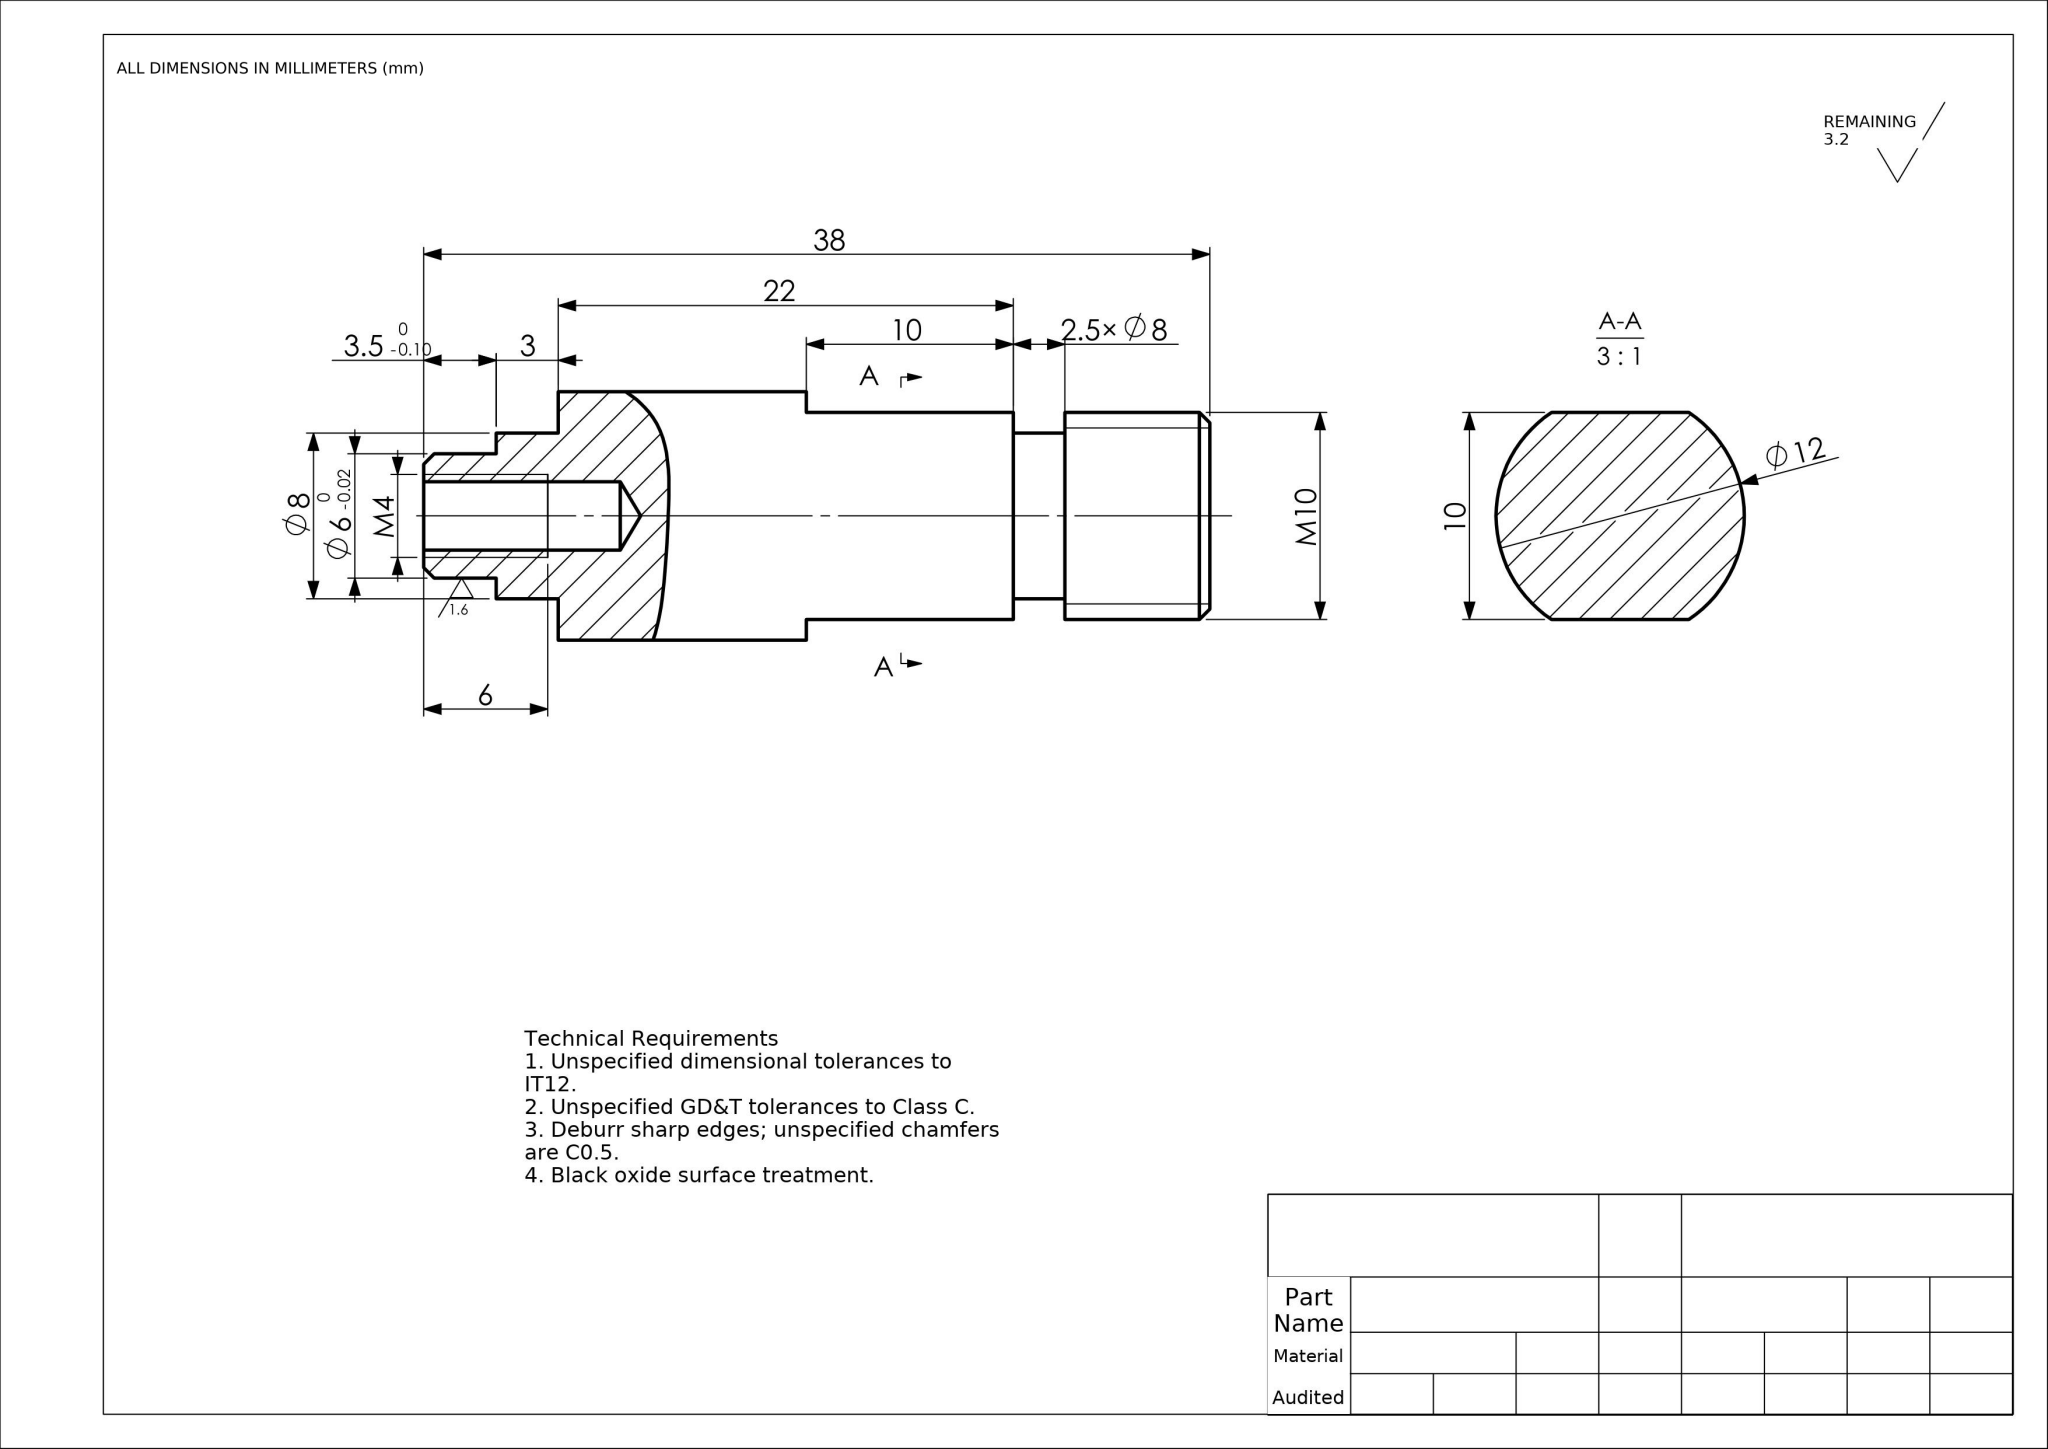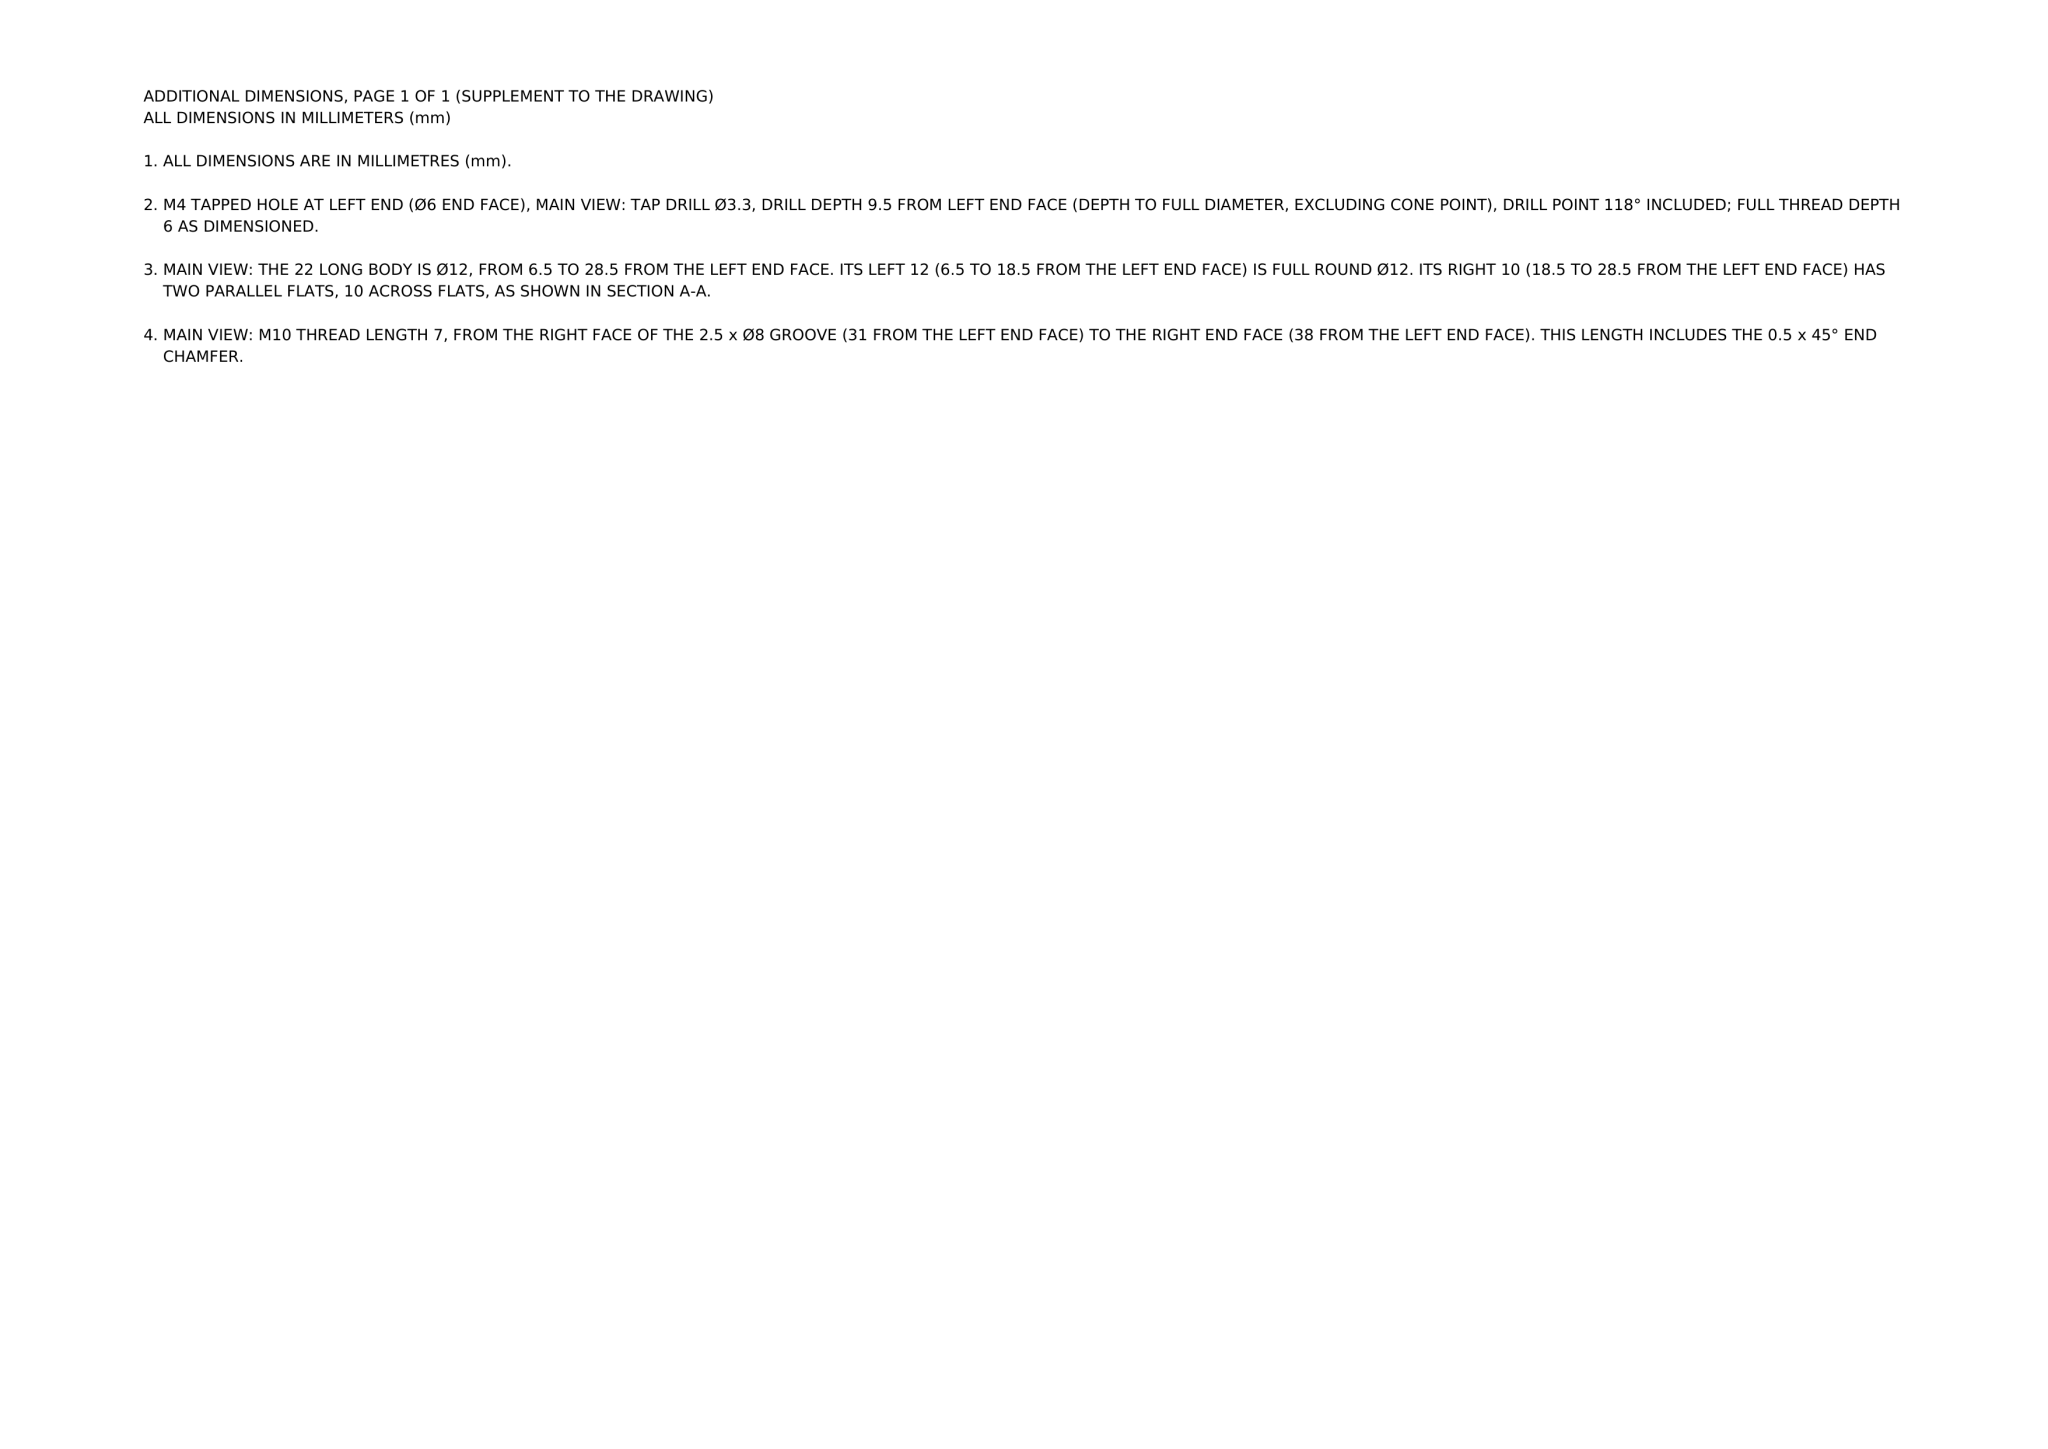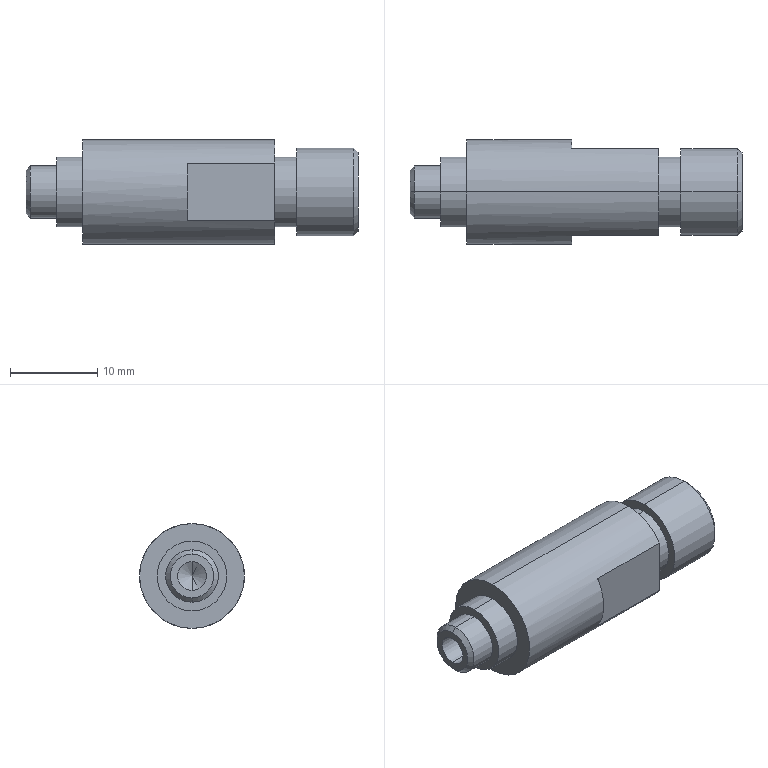Part | NX | mm | 1 solid | 28 faces | box 38 x 12 x 12 mm | volume 3233 mm3 | cylinder 12 | plane 10 | cone 6 | commonest cylinder face diameters 8 x4 3.3 x2 10 x2 12 x2 6 x2
STEP:
#1=COLOUR_RGB('',0.7961,0.8235,0.9373);
#2=FILL_AREA_STYLE_COLOUR('',#1);
#3=FILL_AREA_STYLE('',(#2));
#4=SURFACE_STYLE_FILL_AREA(#3);
#5=SURFACE_SIDE_STYLE('',(#4));
#6=SURFACE_STYLE_USAGE(.BOTH.,#5);
#7=PRESENTATION_STYLE_ASSIGNMENT((#6));
#8=CARTESIAN_POINT('',(9.5,0.,-1.65));
#9=VERTEX_POINT('',#8);
#10=CARTESIAN_POINT('',(9.5,0.,1.65));
#11=VERTEX_POINT('',#10);
#12=CARTESIAN_POINT('',(9.5,0.,0.));
#13=DIRECTION('',(-1.,0.,0.));
#14=DIRECTION('',(0.,0.,1.));
#15=AXIS2_PLACEMENT_3D('',#12,#13,#14);
#16=CIRCLE('',#15,1.65);
#17=EDGE_CURVE('',#9,#11,#16,.T.);
#18=ORIENTED_EDGE('',*,*,#17,.F.);
#19=CARTESIAN_POINT('',(-0.,0.,-1.65));
#20=VERTEX_POINT('',#19);
#21=CARTESIAN_POINT('',(0.,0.,-1.65));
#22=DIRECTION('',(-1.,0.,0.));
#23=VECTOR('',#22,1000.);
#24=LINE('',#21,#23);
#25=EDGE_CURVE('',#9,#20,#24,.T.);
#26=ORIENTED_EDGE('',*,*,#25,.T.);
#27=CARTESIAN_POINT('',(-0.,0.,1.65));
#28=VERTEX_POINT('',#27);
#29=CARTESIAN_POINT('',(-0.,0.,0.));
#30=DIRECTION('',(-1.,0.,0.));
#31=DIRECTION('',(0.,0.,1.));
#32=AXIS2_PLACEMENT_3D('',#29,#30,#31);
#33=CIRCLE('',#32,1.65);
#34=EDGE_CURVE('',#20,#28,#33,.T.);
#35=ORIENTED_EDGE('',*,*,#34,.T.);
#36=CARTESIAN_POINT('',(0.,0.,1.65));
#37=DIRECTION('',(-1.,0.,0.));
#38=VECTOR('',#37,1000.);
#39=LINE('',#36,#38);
#40=EDGE_CURVE('',#11,#28,#39,.T.);
#41=ORIENTED_EDGE('',*,*,#40,.F.);
#42=EDGE_LOOP('',(#18,#26,#35,#41));
#43=FACE_OUTER_BOUND('',#42,.T.);
#44=CARTESIAN_POINT('',(0.,0.,0.));
#45=DIRECTION('',(-1.,0.,0.));
#46=DIRECTION('',(0.,0.,1.));
#47=AXIS2_PLACEMENT_3D('',#44,#45,#46);
#48=CYLINDRICAL_SURFACE('',#47,1.65);
#49=ADVANCED_FACE('',(#43),#48,.F.);
#50=CARTESIAN_POINT('',(10.491,-0.,0.));
#51=VERTEX_POINT('',#50);
#52=CARTESIAN_POINT('',(9.5,0.,1.65));
#53=DIRECTION('',(-0.515,0.,0.8572));
#54=VECTOR('',#53,1000.);
#55=LINE('',#52,#54);
#56=EDGE_CURVE('',#51,#11,#55,.T.);
#57=ORIENTED_EDGE('',*,*,#56,.F.);
#58=CARTESIAN_POINT('',(9.5,0.,-1.65));
#59=DIRECTION('',(-0.515,0.,-0.8572));
#60=VECTOR('',#59,1000.);
#61=LINE('',#58,#60);
#62=EDGE_CURVE('',#51,#9,#61,.T.);
#63=ORIENTED_EDGE('',*,*,#62,.T.);
#64=ORIENTED_EDGE('',*,*,#17,.T.);
#65=EDGE_LOOP('',(#57,#63,#64));
#66=FACE_OUTER_BOUND('',#65,.T.);
#67=CARTESIAN_POINT('',(9.5,0.,0.));
#68=DIRECTION('',(-1.,0.,0.));
#69=DIRECTION('',(0.,0.,1.));
#70=AXIS2_PLACEMENT_3D('',#67,#68,#69);
#71=CONICAL_SURFACE('',#70,1.65,1.03);
#72=ADVANCED_FACE('',(#66),#71,.F.);
#73=CARTESIAN_POINT('',(0.,0.,2.5));
#74=VERTEX_POINT('',#73);
#75=CARTESIAN_POINT('',(0.,0.,-2.5));
#76=VERTEX_POINT('',#75);
#77=CARTESIAN_POINT('',(0.,0.,0.));
#78=DIRECTION('',(-1.,0.,0.));
#79=DIRECTION('',(0.,0.,-1.));
#80=AXIS2_PLACEMENT_3D('',#77,#78,#79);
#81=CIRCLE('',#80,2.5);
#82=EDGE_CURVE('',#74,#76,#81,.T.);
#83=ORIENTED_EDGE('',*,*,#82,.F.);
#84=CARTESIAN_POINT('',(0.5,0.,3.));
#85=VERTEX_POINT('',#84);
#86=CARTESIAN_POINT('',(0.,0.,2.5));
#87=DIRECTION('',(0.7071,0.,0.7071));
#88=VECTOR('',#87,1000.);
#89=LINE('',#86,#88);
#90=EDGE_CURVE('',#74,#85,#89,.T.);
#91=ORIENTED_EDGE('',*,*,#90,.T.);
#92=CARTESIAN_POINT('',(0.5,0.,-3.));
#93=VERTEX_POINT('',#92);
#94=CARTESIAN_POINT('',(0.5,0.,0.));
#95=DIRECTION('',(1.,0.,0.));
#96=DIRECTION('',(0.,0.,-1.));
#97=AXIS2_PLACEMENT_3D('',#94,#95,#96);
#98=CIRCLE('',#97,3.);
#99=EDGE_CURVE('',#93,#85,#98,.T.);
#100=ORIENTED_EDGE('',*,*,#99,.F.);
#101=CARTESIAN_POINT('',(0.,0.,-2.5));
#102=DIRECTION('',(0.7071,0.,-0.7071));
#103=VECTOR('',#102,1000.);
#104=LINE('',#101,#103);
#105=EDGE_CURVE('',#76,#93,#104,.T.);
#106=ORIENTED_EDGE('',*,*,#105,.F.);
#107=EDGE_LOOP('',(#83,#91,#100,#106));
#108=FACE_OUTER_BOUND('',#107,.T.);
#109=CARTESIAN_POINT('',(0.,0.,0.));
#110=DIRECTION('',(1.,0.,0.));
#111=DIRECTION('',(0.,0.,-1.));
#112=AXIS2_PLACEMENT_3D('',#109,#110,#111);
#113=CONICAL_SURFACE('',#112,2.5,0.7854);
#114=ADVANCED_FACE('',(#108),#113,.T.);
#115=CARTESIAN_POINT('',(38.,0.,-4.5));
#116=VERTEX_POINT('',#115);
#117=CARTESIAN_POINT('',(38.,0.,4.5));
#118=VERTEX_POINT('',#117);
#119=CARTESIAN_POINT('',(38.,0.,0.));
#120=DIRECTION('',(1.,0.,0.));
#121=DIRECTION('',(0.,0.,1.));
#122=AXIS2_PLACEMENT_3D('',#119,#120,#121);
#123=CIRCLE('',#122,4.5);
#124=EDGE_CURVE('',#116,#118,#123,.T.);
#125=ORIENTED_EDGE('',*,*,#124,.F.);
#126=CARTESIAN_POINT('',(37.5,0.,-5.));
#127=VERTEX_POINT('',#126);
#128=CARTESIAN_POINT('',(37.5,0.,-5.));
#129=DIRECTION('',(-0.7071,0.,-0.7071));
#130=VECTOR('',#129,1000.);
#131=LINE('',#128,#130);
#132=EDGE_CURVE('',#116,#127,#131,.T.);
#133=ORIENTED_EDGE('',*,*,#132,.T.);
#134=CARTESIAN_POINT('',(37.5,0.,5.));
#135=VERTEX_POINT('',#134);
#136=CARTESIAN_POINT('',(37.5,0.,0.));
#137=DIRECTION('',(-1.,0.,0.));
#138=DIRECTION('',(0.,0.,1.));
#139=AXIS2_PLACEMENT_3D('',#136,#137,#138);
#140=CIRCLE('',#139,5.);
#141=EDGE_CURVE('',#135,#127,#140,.T.);
#142=ORIENTED_EDGE('',*,*,#141,.F.);
#143=CARTESIAN_POINT('',(37.5,0.,5.));
#144=DIRECTION('',(-0.7071,0.,0.7071));
#145=VECTOR('',#144,1000.);
#146=LINE('',#143,#145);
#147=EDGE_CURVE('',#118,#135,#146,.T.);
#148=ORIENTED_EDGE('',*,*,#147,.F.);
#149=EDGE_LOOP('',(#125,#133,#142,#148));
#150=FACE_OUTER_BOUND('',#149,.T.);
#151=CARTESIAN_POINT('',(37.5,0.,0.));
#152=DIRECTION('',(-1.,0.,0.));
#153=DIRECTION('',(0.,0.,1.));
#154=AXIS2_PLACEMENT_3D('',#151,#152,#153);
#155=CONICAL_SURFACE('',#154,5.,0.7854);
#156=ADVANCED_FACE('',(#150),#155,.T.);
#157=ORIENTED_EDGE('',*,*,#141,.T.);
#158=CARTESIAN_POINT('',(31.,0.,-5.));
#159=VERTEX_POINT('',#158);
#160=CARTESIAN_POINT('',(-32.06,0.,-5.));
#161=DIRECTION('',(-1.,0.,0.));
#162=VECTOR('',#161,1000.);
#163=LINE('',#160,#162);
#164=EDGE_CURVE('',#127,#159,#163,.T.);
#165=ORIENTED_EDGE('',*,*,#164,.T.);
#166=CARTESIAN_POINT('',(31.,0.,5.));
#167=VERTEX_POINT('',#166);
#168=CARTESIAN_POINT('',(31.,0.,0.));
#169=DIRECTION('',(-1.,0.,0.));
#170=DIRECTION('',(0.,0.,1.));
#171=AXIS2_PLACEMENT_3D('',#168,#169,#170);
#172=CIRCLE('',#171,5.);
#173=EDGE_CURVE('',#167,#159,#172,.T.);
#174=ORIENTED_EDGE('',*,*,#173,.F.);
#175=CARTESIAN_POINT('',(-32.06,0.,5.));
#176=DIRECTION('',(-1.,0.,0.));
#177=VECTOR('',#176,1000.);
#178=LINE('',#175,#177);
#179=EDGE_CURVE('',#135,#167,#178,.T.);
#180=ORIENTED_EDGE('',*,*,#179,.F.);
#181=EDGE_LOOP('',(#157,#165,#174,#180));
#182=FACE_OUTER_BOUND('',#181,.T.);
#183=CARTESIAN_POINT('',(-32.06,0.,0.));
#184=DIRECTION('',(-1.,0.,0.));
#185=DIRECTION('',(0.,0.,1.));
#186=AXIS2_PLACEMENT_3D('',#183,#184,#185);
#187=CYLINDRICAL_SURFACE('',#186,5.);
#188=ADVANCED_FACE('',(#182),#187,.T.);
#189=CARTESIAN_POINT('',(31.,0.,4.));
#190=VERTEX_POINT('',#189);
#191=CARTESIAN_POINT('',(31.,0.,-4.));
#192=VERTEX_POINT('',#191);
#193=CARTESIAN_POINT('',(31.,0.,0.));
#194=DIRECTION('',(-1.,0.,0.));
#195=DIRECTION('',(0.,0.,1.));
#196=AXIS2_PLACEMENT_3D('',#193,#194,#195);
#197=CIRCLE('',#196,4.);
#198=EDGE_CURVE('',#190,#192,#197,.T.);
#199=ORIENTED_EDGE('',*,*,#198,.T.);
#200=CARTESIAN_POINT('',(28.5,0.,-4.));
#201=VERTEX_POINT('',#200);
#202=CARTESIAN_POINT('',(-32.06,0.,-4.));
#203=DIRECTION('',(-1.,0.,0.));
#204=VECTOR('',#203,1000.);
#205=LINE('',#202,#204);
#206=EDGE_CURVE('',#192,#201,#205,.T.);
#207=ORIENTED_EDGE('',*,*,#206,.T.);
#208=CARTESIAN_POINT('',(28.5,0.,4.));
#209=VERTEX_POINT('',#208);
#210=CARTESIAN_POINT('',(28.5,0.,0.));
#211=DIRECTION('',(-1.,0.,0.));
#212=DIRECTION('',(0.,0.,1.));
#213=AXIS2_PLACEMENT_3D('',#210,#211,#212);
#214=CIRCLE('',#213,4.);
#215=EDGE_CURVE('',#209,#201,#214,.T.);
#216=ORIENTED_EDGE('',*,*,#215,.F.);
#217=CARTESIAN_POINT('',(-32.06,0.,4.));
#218=DIRECTION('',(-1.,0.,0.));
#219=VECTOR('',#218,1000.);
#220=LINE('',#217,#219);
#221=EDGE_CURVE('',#190,#209,#220,.T.);
#222=ORIENTED_EDGE('',*,*,#221,.F.);
#223=EDGE_LOOP('',(#199,#207,#216,#222));
#224=FACE_OUTER_BOUND('',#223,.T.);
#225=CARTESIAN_POINT('',(-32.06,0.,0.));
#226=DIRECTION('',(-1.,0.,0.));
#227=DIRECTION('',(0.,0.,1.));
#228=AXIS2_PLACEMENT_3D('',#225,#226,#227);
#229=CYLINDRICAL_SURFACE('',#228,4.);
#230=ADVANCED_FACE('',(#224),#229,.T.);
#231=CARTESIAN_POINT('',(28.5,5.,-3.317));
#232=VERTEX_POINT('',#231);
#233=CARTESIAN_POINT('',(28.5,0.,-6.));
#234=VERTEX_POINT('',#233);
#235=CARTESIAN_POINT('',(28.5,0.,0.));
#236=DIRECTION('',(-1.,0.,0.));
#237=DIRECTION('',(0.,0.,1.));
#238=AXIS2_PLACEMENT_3D('',#235,#236,#237);
#239=CIRCLE('',#238,6.);
#240=EDGE_CURVE('',#232,#234,#239,.T.);
#241=ORIENTED_EDGE('',*,*,#240,.T.);
#242=CARTESIAN_POINT('',(6.5,0.,-6.));
#243=VERTEX_POINT('',#242);
#244=CARTESIAN_POINT('',(-32.06,0.,-6.));
#245=DIRECTION('',(-1.,0.,0.));
#246=VECTOR('',#245,1000.);
#247=LINE('',#244,#246);
#248=EDGE_CURVE('',#234,#243,#247,.T.);
#249=ORIENTED_EDGE('',*,*,#248,.T.);
#250=CARTESIAN_POINT('',(6.5,0.,6.));
#251=VERTEX_POINT('',#250);
#252=CARTESIAN_POINT('',(6.5,0.,0.));
#253=DIRECTION('',(-1.,0.,0.));
#254=DIRECTION('',(0.,0.,1.));
#255=AXIS2_PLACEMENT_3D('',#252,#253,#254);
#256=CIRCLE('',#255,6.);
#257=EDGE_CURVE('',#251,#243,#256,.T.);
#258=ORIENTED_EDGE('',*,*,#257,.F.);
#259=CARTESIAN_POINT('',(28.5,0.,6.));
#260=VERTEX_POINT('',#259);
#261=CARTESIAN_POINT('',(-32.06,0.,6.));
#262=DIRECTION('',(-1.,0.,0.));
#263=VECTOR('',#262,1000.);
#264=LINE('',#261,#263);
#265=EDGE_CURVE('',#260,#251,#264,.T.);
#266=ORIENTED_EDGE('',*,*,#265,.F.);
#267=CARTESIAN_POINT('',(28.5,5.,3.317));
#268=VERTEX_POINT('',#267);
#269=CARTESIAN_POINT('',(28.5,0.,0.));
#270=DIRECTION('',(-1.,0.,0.));
#271=DIRECTION('',(0.,0.,1.));
#272=AXIS2_PLACEMENT_3D('',#269,#270,#271);
#273=CIRCLE('',#272,6.);
#274=EDGE_CURVE('',#260,#268,#273,.T.);
#275=ORIENTED_EDGE('',*,*,#274,.T.);
#276=CARTESIAN_POINT('',(18.5,5.,3.317));
#277=VERTEX_POINT('',#276);
#278=CARTESIAN_POINT('',(-32.06,5.,3.317));
#279=DIRECTION('',(-1.,0.,0.));
#280=VECTOR('',#279,1000.);
#281=LINE('',#278,#280);
#282=EDGE_CURVE('',#268,#277,#281,.T.);
#283=ORIENTED_EDGE('',*,*,#282,.T.);
#284=CARTESIAN_POINT('',(18.5,5.,-3.317));
#285=VERTEX_POINT('',#284);
#286=CARTESIAN_POINT('',(18.5,0.,0.));
#287=DIRECTION('',(-1.,0.,0.));
#288=DIRECTION('',(0.,0.,1.));
#289=AXIS2_PLACEMENT_3D('',#286,#287,#288);
#290=CIRCLE('',#289,6.);
#291=EDGE_CURVE('',#277,#285,#290,.T.);
#292=ORIENTED_EDGE('',*,*,#291,.T.);
#293=CARTESIAN_POINT('',(-32.06,5.,-3.317));
#294=DIRECTION('',(1.,0.,0.));
#295=VECTOR('',#294,1000.);
#296=LINE('',#293,#295);
#297=EDGE_CURVE('',#285,#232,#296,.T.);
#298=ORIENTED_EDGE('',*,*,#297,.T.);
#299=EDGE_LOOP('',(#241,#249,#258,#266,#275,#283,#292,#298));
#300=FACE_OUTER_BOUND('',#299,.T.);
#301=CARTESIAN_POINT('',(-32.06,0.,0.));
#302=DIRECTION('',(-1.,0.,0.));
#303=DIRECTION('',(0.,0.,1.));
#304=AXIS2_PLACEMENT_3D('',#301,#302,#303);
#305=CYLINDRICAL_SURFACE('',#304,6.);
#306=ADVANCED_FACE('',(#300),#305,.T.);
#307=CARTESIAN_POINT('',(6.5,0.,4.));
#308=VERTEX_POINT('',#307);
#309=CARTESIAN_POINT('',(6.5,0.,-4.));
#310=VERTEX_POINT('',#309);
#311=CARTESIAN_POINT('',(6.5,0.,0.));
#312=DIRECTION('',(-1.,0.,0.));
#313=DIRECTION('',(0.,0.,1.));
#314=AXIS2_PLACEMENT_3D('',#311,#312,#313);
#315=CIRCLE('',#314,4.);
#316=EDGE_CURVE('',#308,#310,#315,.T.);
#317=ORIENTED_EDGE('',*,*,#316,.T.);
#318=CARTESIAN_POINT('',(3.5,0.,-4.));
#319=VERTEX_POINT('',#318);
#320=CARTESIAN_POINT('',(-32.06,0.,-4.));
#321=DIRECTION('',(-1.,0.,0.));
#322=VECTOR('',#321,1000.);
#323=LINE('',#320,#322);
#324=EDGE_CURVE('',#310,#319,#323,.T.);
#325=ORIENTED_EDGE('',*,*,#324,.T.);
#326=CARTESIAN_POINT('',(3.5,0.,4.));
#327=VERTEX_POINT('',#326);
#328=CARTESIAN_POINT('',(3.5,0.,0.));
#329=DIRECTION('',(-1.,0.,0.));
#330=DIRECTION('',(0.,0.,1.));
#331=AXIS2_PLACEMENT_3D('',#328,#329,#330);
#332=CIRCLE('',#331,4.);
#333=EDGE_CURVE('',#327,#319,#332,.T.);
#334=ORIENTED_EDGE('',*,*,#333,.F.);
#335=CARTESIAN_POINT('',(-32.06,0.,4.));
#336=DIRECTION('',(-1.,0.,0.));
#337=VECTOR('',#336,1000.);
#338=LINE('',#335,#337);
#339=EDGE_CURVE('',#308,#327,#338,.T.);
#340=ORIENTED_EDGE('',*,*,#339,.F.);
#341=EDGE_LOOP('',(#317,#325,#334,#340));
#342=FACE_OUTER_BOUND('',#341,.T.);
#343=CARTESIAN_POINT('',(-32.06,0.,0.));
#344=DIRECTION('',(-1.,0.,0.));
#345=DIRECTION('',(0.,0.,1.));
#346=AXIS2_PLACEMENT_3D('',#343,#344,#345);
#347=CYLINDRICAL_SURFACE('',#346,4.);
#348=ADVANCED_FACE('',(#342),#347,.T.);
#349=CARTESIAN_POINT('',(3.5,0.,3.));
#350=VERTEX_POINT('',#349);
#351=CARTESIAN_POINT('',(3.5,0.,-3.));
#352=VERTEX_POINT('',#351);
#353=CARTESIAN_POINT('',(3.5,0.,0.));
#354=DIRECTION('',(-1.,0.,0.));
#355=DIRECTION('',(0.,0.,1.));
#356=AXIS2_PLACEMENT_3D('',#353,#354,#355);
#357=CIRCLE('',#356,3.);
#358=EDGE_CURVE('',#350,#352,#357,.T.);
#359=ORIENTED_EDGE('',*,*,#358,.T.);
#360=CARTESIAN_POINT('',(-32.06,0.,-3.));
#361=DIRECTION('',(-1.,0.,0.));
#362=VECTOR('',#361,1000.);
#363=LINE('',#360,#362);
#364=EDGE_CURVE('',#352,#93,#363,.T.);
#365=ORIENTED_EDGE('',*,*,#364,.T.);
#366=ORIENTED_EDGE('',*,*,#99,.T.);
#367=CARTESIAN_POINT('',(-32.06,0.,3.));
#368=DIRECTION('',(-1.,0.,0.));
#369=VECTOR('',#368,1000.);
#370=LINE('',#367,#369);
#371=EDGE_CURVE('',#350,#85,#370,.T.);
#372=ORIENTED_EDGE('',*,*,#371,.F.);
#373=EDGE_LOOP('',(#359,#365,#366,#372));
#374=FACE_OUTER_BOUND('',#373,.T.);
#375=CARTESIAN_POINT('',(-32.06,0.,0.));
#376=DIRECTION('',(-1.,0.,0.));
#377=DIRECTION('',(0.,0.,1.));
#378=AXIS2_PLACEMENT_3D('',#375,#376,#377);
#379=CYLINDRICAL_SURFACE('',#378,3.);
#380=ADVANCED_FACE('',(#374),#379,.T.);
#381=CARTESIAN_POINT('',(-0.,0.,0.));
#382=DIRECTION('',(-1.,0.,0.));
#383=DIRECTION('',(0.,0.,1.));
#384=AXIS2_PLACEMENT_3D('',#381,#382,#383);
#385=CIRCLE('',#384,1.65);
#386=EDGE_CURVE('',#28,#20,#385,.T.);
#387=ORIENTED_EDGE('',*,*,#386,.F.);
#388=ORIENTED_EDGE('',*,*,#34,.F.);
#389=EDGE_LOOP('',(#387,#388));
#390=FACE_BOUND('',#389,.T.);
#391=CARTESIAN_POINT('',(0.,0.,0.));
#392=DIRECTION('',(-1.,0.,0.));
#393=DIRECTION('',(0.,0.,-1.));
#394=AXIS2_PLACEMENT_3D('',#391,#392,#393);
#395=CIRCLE('',#394,2.5);
#396=EDGE_CURVE('',#76,#74,#395,.T.);
#397=ORIENTED_EDGE('',*,*,#396,.T.);
#398=ORIENTED_EDGE('',*,*,#82,.T.);
#399=EDGE_LOOP('',(#397,#398));
#400=FACE_OUTER_BOUND('',#399,.T.);
#401=CARTESIAN_POINT('',(0.,0.,0.));
#402=DIRECTION('',(1.,0.,0.));
#403=DIRECTION('',(0.,0.,-1.));
#404=AXIS2_PLACEMENT_3D('',#401,#402,#403);
#405=PLANE('',#404);
#406=ADVANCED_FACE('',(#390,#400),#405,.F.);
#407=ORIENTED_EDGE('',*,*,#364,.F.);
#408=CARTESIAN_POINT('',(3.5,0.,0.));
#409=DIRECTION('',(-1.,0.,0.));
#410=DIRECTION('',(0.,0.,1.));
#411=AXIS2_PLACEMENT_3D('',#408,#409,#410);
#412=CIRCLE('',#411,3.);
#413=EDGE_CURVE('',#352,#350,#412,.T.);
#414=ORIENTED_EDGE('',*,*,#413,.T.);
#415=ORIENTED_EDGE('',*,*,#371,.T.);
#416=CARTESIAN_POINT('',(0.5,0.,0.));
#417=DIRECTION('',(1.,0.,0.));
#418=DIRECTION('',(0.,0.,-1.));
#419=AXIS2_PLACEMENT_3D('',#416,#417,#418);
#420=CIRCLE('',#419,3.);
#421=EDGE_CURVE('',#85,#93,#420,.T.);
#422=ORIENTED_EDGE('',*,*,#421,.T.);
#423=EDGE_LOOP('',(#407,#414,#415,#422));
#424=FACE_OUTER_BOUND('',#423,.T.);
#425=CARTESIAN_POINT('',(-32.06,0.,0.));
#426=DIRECTION('',(-1.,0.,0.));
#427=DIRECTION('',(0.,0.,1.));
#428=AXIS2_PLACEMENT_3D('',#425,#426,#427);
#429=CYLINDRICAL_SURFACE('',#428,3.);
#430=ADVANCED_FACE('',(#424),#429,.T.);
#431=ORIENTED_EDGE('',*,*,#358,.F.);
#432=ORIENTED_EDGE('',*,*,#413,.F.);
#433=EDGE_LOOP('',(#431,#432));
#434=FACE_BOUND('',#433,.T.);
#435=ORIENTED_EDGE('',*,*,#333,.T.);
#436=CARTESIAN_POINT('',(3.5,0.,0.));
#437=DIRECTION('',(-1.,0.,0.));
#438=DIRECTION('',(0.,0.,1.));
#439=AXIS2_PLACEMENT_3D('',#436,#437,#438);
#440=CIRCLE('',#439,4.);
#441=EDGE_CURVE('',#319,#327,#440,.T.);
#442=ORIENTED_EDGE('',*,*,#441,.T.);
#443=EDGE_LOOP('',(#435,#442));
#444=FACE_OUTER_BOUND('',#443,.T.);
#445=CARTESIAN_POINT('',(3.5,3.,0.));
#446=DIRECTION('',(1.,0.,0.));
#447=DIRECTION('',(0.,0.,-1.));
#448=AXIS2_PLACEMENT_3D('',#445,#446,#447);
#449=PLANE('',#448);
#450=ADVANCED_FACE('',(#434,#444),#449,.F.);
#451=ORIENTED_EDGE('',*,*,#324,.F.);
#452=CARTESIAN_POINT('',(6.5,0.,0.));
#453=DIRECTION('',(-1.,0.,0.));
#454=DIRECTION('',(0.,0.,1.));
#455=AXIS2_PLACEMENT_3D('',#452,#453,#454);
#456=CIRCLE('',#455,4.);
#457=EDGE_CURVE('',#310,#308,#456,.T.);
#458=ORIENTED_EDGE('',*,*,#457,.T.);
#459=ORIENTED_EDGE('',*,*,#339,.T.);
#460=ORIENTED_EDGE('',*,*,#441,.F.);
#461=EDGE_LOOP('',(#451,#458,#459,#460));
#462=FACE_OUTER_BOUND('',#461,.T.);
#463=CARTESIAN_POINT('',(-32.06,0.,0.));
#464=DIRECTION('',(-1.,0.,0.));
#465=DIRECTION('',(0.,0.,1.));
#466=AXIS2_PLACEMENT_3D('',#463,#464,#465);
#467=CYLINDRICAL_SURFACE('',#466,4.);
#468=ADVANCED_FACE('',(#462),#467,.T.);
#469=ORIENTED_EDGE('',*,*,#316,.F.);
#470=ORIENTED_EDGE('',*,*,#457,.F.);
#471=EDGE_LOOP('',(#469,#470));
#472=FACE_BOUND('',#471,.T.);
#473=ORIENTED_EDGE('',*,*,#257,.T.);
#474=CARTESIAN_POINT('',(6.5,0.,0.));
#475=DIRECTION('',(-1.,0.,0.));
#476=DIRECTION('',(0.,0.,1.));
#477=AXIS2_PLACEMENT_3D('',#474,#475,#476);
#478=CIRCLE('',#477,6.);
#479=EDGE_CURVE('',#243,#251,#478,.T.);
#480=ORIENTED_EDGE('',*,*,#479,.T.);
#481=EDGE_LOOP('',(#473,#480));
#482=FACE_OUTER_BOUND('',#481,.T.);
#483=CARTESIAN_POINT('',(6.5,4.,0.));
#484=DIRECTION('',(1.,0.,0.));
#485=DIRECTION('',(0.,0.,-1.));
#486=AXIS2_PLACEMENT_3D('',#483,#484,#485);
#487=PLANE('',#486);
#488=ADVANCED_FACE('',(#472,#482),#487,.F.);
#489=ORIENTED_EDGE('',*,*,#248,.F.);
#490=CARTESIAN_POINT('',(28.5,-5.,-3.317));
#491=VERTEX_POINT('',#490);
#492=CARTESIAN_POINT('',(28.5,0.,0.));
#493=DIRECTION('',(-1.,0.,0.));
#494=DIRECTION('',(0.,0.,1.));
#495=AXIS2_PLACEMENT_3D('',#492,#493,#494);
#496=CIRCLE('',#495,6.);
#497=EDGE_CURVE('',#234,#491,#496,.T.);
#498=ORIENTED_EDGE('',*,*,#497,.T.);
#499=CARTESIAN_POINT('',(18.5,-5.,-3.317));
#500=VERTEX_POINT('',#499);
#501=CARTESIAN_POINT('',(-32.06,-5.,-3.317));
#502=DIRECTION('',(-1.,0.,0.));
#503=VECTOR('',#502,1000.);
#504=LINE('',#501,#503);
#505=EDGE_CURVE('',#491,#500,#504,.T.);
#506=ORIENTED_EDGE('',*,*,#505,.T.);
#507=CARTESIAN_POINT('',(18.5,-5.,3.317));
#508=VERTEX_POINT('',#507);
#509=CARTESIAN_POINT('',(18.5,0.,0.));
#510=DIRECTION('',(-1.,0.,0.));
#511=DIRECTION('',(-0.,-1.,0.));
#512=AXIS2_PLACEMENT_3D('',#509,#510,#511);
#513=CIRCLE('',#512,6.);
#514=EDGE_CURVE('',#500,#508,#513,.T.);
#515=ORIENTED_EDGE('',*,*,#514,.T.);
#516=CARTESIAN_POINT('',(28.5,-5.,3.317));
#517=VERTEX_POINT('',#516);
#518=CARTESIAN_POINT('',(-32.06,-5.,3.317));
#519=DIRECTION('',(1.,0.,0.));
#520=VECTOR('',#519,1000.);
#521=LINE('',#518,#520);
#522=EDGE_CURVE('',#508,#517,#521,.T.);
#523=ORIENTED_EDGE('',*,*,#522,.T.);
#524=CARTESIAN_POINT('',(28.5,0.,0.));
#525=DIRECTION('',(-1.,0.,0.));
#526=DIRECTION('',(0.,0.,1.));
#527=AXIS2_PLACEMENT_3D('',#524,#525,#526);
#528=CIRCLE('',#527,6.);
#529=EDGE_CURVE('',#517,#260,#528,.T.);
#530=ORIENTED_EDGE('',*,*,#529,.T.);
#531=ORIENTED_EDGE('',*,*,#265,.T.);
#532=ORIENTED_EDGE('',*,*,#479,.F.);
#533=EDGE_LOOP('',(#489,#498,#506,#515,#523,#530,#531,#532));
#534=FACE_OUTER_BOUND('',#533,.T.);
#535=CARTESIAN_POINT('',(-32.06,0.,0.));
#536=DIRECTION('',(-1.,0.,0.));
#537=DIRECTION('',(0.,0.,1.));
#538=AXIS2_PLACEMENT_3D('',#535,#536,#537);
#539=CYLINDRICAL_SURFACE('',#538,6.);
#540=ADVANCED_FACE('',(#534),#539,.T.);
#541=ORIENTED_EDGE('',*,*,#529,.F.);
#542=CARTESIAN_POINT('',(28.5,-5.,0.));
#543=DIRECTION('',(0.,0.,-1.));
#544=VECTOR('',#543,1000.);
#545=LINE('',#542,#544);
#546=EDGE_CURVE('',#517,#491,#545,.T.);
#547=ORIENTED_EDGE('',*,*,#546,.T.);
#548=ORIENTED_EDGE('',*,*,#497,.F.);
#549=ORIENTED_EDGE('',*,*,#240,.F.);
#550=CARTESIAN_POINT('',(28.5,5.,0.));
#551=DIRECTION('',(0.,0.,1.));
#552=VECTOR('',#551,1000.);
#553=LINE('',#550,#552);
#554=EDGE_CURVE('',#232,#268,#553,.T.);
#555=ORIENTED_EDGE('',*,*,#554,.T.);
#556=ORIENTED_EDGE('',*,*,#274,.F.);
#557=EDGE_LOOP('',(#541,#547,#548,#549,#555,#556));
#558=FACE_OUTER_BOUND('',#557,.T.);
#559=ORIENTED_EDGE('',*,*,#215,.T.);
#560=CARTESIAN_POINT('',(28.5,0.,0.));
#561=DIRECTION('',(-1.,0.,0.));
#562=DIRECTION('',(0.,0.,1.));
#563=AXIS2_PLACEMENT_3D('',#560,#561,#562);
#564=CIRCLE('',#563,4.);
#565=EDGE_CURVE('',#201,#209,#564,.T.);
#566=ORIENTED_EDGE('',*,*,#565,.T.);
#567=EDGE_LOOP('',(#559,#566));
#568=FACE_BOUND('',#567,.T.);
#569=CARTESIAN_POINT('',(28.5,6.,0.));
#570=DIRECTION('',(-1.,0.,0.));
#571=DIRECTION('',(0.,0.,1.));
#572=AXIS2_PLACEMENT_3D('',#569,#570,#571);
#573=PLANE('',#572);
#574=ADVANCED_FACE('',(#558,#568),#573,.F.);
#575=ORIENTED_EDGE('',*,*,#206,.F.);
#576=CARTESIAN_POINT('',(31.,0.,0.));
#577=DIRECTION('',(-1.,0.,0.));
#578=DIRECTION('',(0.,0.,1.));
#579=AXIS2_PLACEMENT_3D('',#576,#577,#578);
#580=CIRCLE('',#579,4.);
#581=EDGE_CURVE('',#192,#190,#580,.T.);
#582=ORIENTED_EDGE('',*,*,#581,.T.);
#583=ORIENTED_EDGE('',*,*,#221,.T.);
#584=ORIENTED_EDGE('',*,*,#565,.F.);
#585=EDGE_LOOP('',(#575,#582,#583,#584));
#586=FACE_OUTER_BOUND('',#585,.T.);
#587=CARTESIAN_POINT('',(-32.06,0.,0.));
#588=DIRECTION('',(-1.,0.,0.));
#589=DIRECTION('',(0.,0.,1.));
#590=AXIS2_PLACEMENT_3D('',#587,#588,#589);
#591=CYLINDRICAL_SURFACE('',#590,4.);
#592=ADVANCED_FACE('',(#586),#591,.T.);
#593=ORIENTED_EDGE('',*,*,#198,.F.);
#594=ORIENTED_EDGE('',*,*,#581,.F.);
#595=EDGE_LOOP('',(#593,#594));
#596=FACE_BOUND('',#595,.T.);
#597=ORIENTED_EDGE('',*,*,#173,.T.);
#598=CARTESIAN_POINT('',(31.,0.,0.));
#599=DIRECTION('',(-1.,0.,0.));
#600=DIRECTION('',(0.,0.,1.));
#601=AXIS2_PLACEMENT_3D('',#598,#599,#600);
#602=CIRCLE('',#601,5.);
#603=EDGE_CURVE('',#159,#167,#602,.T.);
#604=ORIENTED_EDGE('',*,*,#603,.T.);
#605=EDGE_LOOP('',(#597,#604));
#606=FACE_OUTER_BOUND('',#605,.T.);
#607=CARTESIAN_POINT('',(31.,4.,0.));
#608=DIRECTION('',(1.,0.,0.));
#609=DIRECTION('',(0.,0.,-1.));
#610=AXIS2_PLACEMENT_3D('',#607,#608,#609);
#611=PLANE('',#610);
#612=ADVANCED_FACE('',(#596,#606),#611,.F.);
#613=ORIENTED_EDGE('',*,*,#164,.F.);
#614=CARTESIAN_POINT('',(37.5,0.,0.));
#615=DIRECTION('',(-1.,0.,0.));
#616=DIRECTION('',(0.,0.,1.));
#617=AXIS2_PLACEMENT_3D('',#614,#615,#616);
#618=CIRCLE('',#617,5.);
#619=EDGE_CURVE('',#127,#135,#618,.T.);
#620=ORIENTED_EDGE('',*,*,#619,.T.);
#621=ORIENTED_EDGE('',*,*,#179,.T.);
#622=ORIENTED_EDGE('',*,*,#603,.F.);
#623=EDGE_LOOP('',(#613,#620,#621,#622));
#624=FACE_OUTER_BOUND('',#623,.T.);
#625=CARTESIAN_POINT('',(-32.06,0.,0.));
#626=DIRECTION('',(-1.,0.,0.));
#627=DIRECTION('',(0.,0.,1.));
#628=AXIS2_PLACEMENT_3D('',#625,#626,#627);
#629=CYLINDRICAL_SURFACE('',#628,5.);
#630=ADVANCED_FACE('',(#624),#629,.T.);
#631=CARTESIAN_POINT('',(38.,0.,0.));
#632=DIRECTION('',(1.,0.,0.));
#633=DIRECTION('',(0.,0.,1.));
#634=AXIS2_PLACEMENT_3D('',#631,#632,#633);
#635=CIRCLE('',#634,4.5);
#636=EDGE_CURVE('',#118,#116,#635,.T.);
#637=ORIENTED_EDGE('',*,*,#636,.T.);
#638=ORIENTED_EDGE('',*,*,#124,.T.);
#639=EDGE_LOOP('',(#637,#638));
#640=FACE_OUTER_BOUND('',#639,.T.);
#641=CARTESIAN_POINT('',(38.,5.,0.));
#642=DIRECTION('',(-1.,0.,0.));
#643=DIRECTION('',(0.,0.,1.));
#644=AXIS2_PLACEMENT_3D('',#641,#642,#643);
#645=PLANE('',#644);
#646=ADVANCED_FACE('',(#640),#645,.F.);
#647=ORIENTED_EDGE('',*,*,#132,.F.);
#648=ORIENTED_EDGE('',*,*,#636,.F.);
#649=ORIENTED_EDGE('',*,*,#147,.T.);
#650=ORIENTED_EDGE('',*,*,#619,.F.);
#651=EDGE_LOOP('',(#647,#648,#649,#650));
#652=FACE_OUTER_BOUND('',#651,.T.);
#653=CARTESIAN_POINT('',(37.5,0.,0.));
#654=DIRECTION('',(-1.,0.,0.));
#655=DIRECTION('',(0.,0.,1.));
#656=AXIS2_PLACEMENT_3D('',#653,#654,#655);
#657=CONICAL_SURFACE('',#656,5.,0.7854);
#658=ADVANCED_FACE('',(#652),#657,.T.);
#659=ORIENTED_EDGE('',*,*,#90,.F.);
#660=ORIENTED_EDGE('',*,*,#396,.F.);
#661=ORIENTED_EDGE('',*,*,#105,.T.);
#662=ORIENTED_EDGE('',*,*,#421,.F.);
#663=EDGE_LOOP('',(#659,#660,#661,#662));
#664=FACE_OUTER_BOUND('',#663,.T.);
#665=CARTESIAN_POINT('',(0.,0.,0.));
#666=DIRECTION('',(1.,0.,0.));
#667=DIRECTION('',(0.,0.,-1.));
#668=AXIS2_PLACEMENT_3D('',#665,#666,#667);
#669=CONICAL_SURFACE('',#668,2.5,0.7854);
#670=ADVANCED_FACE('',(#664),#669,.T.);
#671=ORIENTED_EDGE('',*,*,#62,.F.);
#672=ORIENTED_EDGE('',*,*,#56,.T.);
#673=CARTESIAN_POINT('',(9.5,0.,0.));
#674=DIRECTION('',(-1.,0.,0.));
#675=DIRECTION('',(0.,0.,1.));
#676=AXIS2_PLACEMENT_3D('',#673,#674,#675);
#677=CIRCLE('',#676,1.65);
#678=EDGE_CURVE('',#11,#9,#677,.T.);
#679=ORIENTED_EDGE('',*,*,#678,.T.);
#680=EDGE_LOOP('',(#671,#672,#679));
#681=FACE_OUTER_BOUND('',#680,.T.);
#682=CARTESIAN_POINT('',(9.5,0.,0.));
#683=DIRECTION('',(-1.,0.,0.));
#684=DIRECTION('',(0.,0.,1.));
#685=AXIS2_PLACEMENT_3D('',#682,#683,#684);
#686=CONICAL_SURFACE('',#685,1.65,1.03);
#687=ADVANCED_FACE('',(#681),#686,.F.);
#688=ORIENTED_EDGE('',*,*,#25,.F.);
#689=ORIENTED_EDGE('',*,*,#678,.F.);
#690=ORIENTED_EDGE('',*,*,#40,.T.);
#691=ORIENTED_EDGE('',*,*,#386,.T.);
#692=EDGE_LOOP('',(#688,#689,#690,#691));
#693=FACE_OUTER_BOUND('',#692,.T.);
#694=CARTESIAN_POINT('',(0.,0.,0.));
#695=DIRECTION('',(-1.,0.,0.));
#696=DIRECTION('',(0.,0.,1.));
#697=AXIS2_PLACEMENT_3D('',#694,#695,#696);
#698=CYLINDRICAL_SURFACE('',#697,1.65);
#699=ADVANCED_FACE('',(#693),#698,.F.);
#700=CARTESIAN_POINT('',(18.5,5.,-5.));
#701=DIRECTION('',(0.,0.,1.));
#702=VECTOR('',#701,1000.);
#703=LINE('',#700,#702);
#704=EDGE_CURVE('',#285,#277,#703,.T.);
#705=ORIENTED_EDGE('',*,*,#704,.F.);
#706=ORIENTED_EDGE('',*,*,#291,.F.);
#707=EDGE_LOOP('',(#705,#706));
#708=FACE_OUTER_BOUND('',#707,.T.);
#709=CARTESIAN_POINT('',(18.5,6.,-5.));
#710=DIRECTION('',(-1.,0.,0.));
#711=DIRECTION('',(0.,0.,1.));
#712=AXIS2_PLACEMENT_3D('',#709,#710,#711);
#713=PLANE('',#712);
#714=ADVANCED_FACE('',(#708),#713,.F.);
#715=ORIENTED_EDGE('',*,*,#554,.F.);
#716=ORIENTED_EDGE('',*,*,#297,.F.);
#717=ORIENTED_EDGE('',*,*,#704,.T.);
#718=ORIENTED_EDGE('',*,*,#282,.F.);
#719=EDGE_LOOP('',(#715,#716,#717,#718));
#720=FACE_OUTER_BOUND('',#719,.T.);
#721=CARTESIAN_POINT('',(18.5,5.,-5.));
#722=DIRECTION('',(0.,-1.,0.));
#723=DIRECTION('',(0.,0.,-1.));
#724=AXIS2_PLACEMENT_3D('',#721,#722,#723);
#725=PLANE('',#724);
#726=ADVANCED_FACE('',(#720),#725,.F.);
#727=ORIENTED_EDGE('',*,*,#514,.F.);
#728=CARTESIAN_POINT('',(18.5,-5.,-5.));
#729=DIRECTION('',(0.,0.,1.));
#730=VECTOR('',#729,1000.);
#731=LINE('',#728,#730);
#732=EDGE_CURVE('',#500,#508,#731,.T.);
#733=ORIENTED_EDGE('',*,*,#732,.T.);
#734=EDGE_LOOP('',(#727,#733));
#735=FACE_OUTER_BOUND('',#734,.T.);
#736=CARTESIAN_POINT('',(18.5,-6.,-5.));
#737=DIRECTION('',(-1.,0.,0.));
#738=DIRECTION('',(-0.,-1.,0.));
#739=AXIS2_PLACEMENT_3D('',#736,#737,#738);
#740=PLANE('',#739);
#741=ADVANCED_FACE('',(#735),#740,.F.);
#742=ORIENTED_EDGE('',*,*,#546,.F.);
#743=ORIENTED_EDGE('',*,*,#522,.F.);
#744=ORIENTED_EDGE('',*,*,#732,.F.);
#745=ORIENTED_EDGE('',*,*,#505,.F.);
#746=EDGE_LOOP('',(#742,#743,#744,#745));
#747=FACE_OUTER_BOUND('',#746,.T.);
#748=CARTESIAN_POINT('',(18.5,-5.,-5.));
#749=DIRECTION('',(0.,1.,0.));
#750=DIRECTION('',(0.,0.,1.));
#751=AXIS2_PLACEMENT_3D('',#748,#749,#750);
#752=PLANE('',#751);
#753=ADVANCED_FACE('',(#747),#752,.F.);
#754=CLOSED_SHELL('',(#49,#72,#114,#156,#188,#230,#306,#348,#380,#406,#430,#450,#468,#488,#540,#574,#592,#612,#630,#646,#658,#670,#687,#699,#714,#726,#741,#753));
#755=MANIFOLD_SOLID_BREP('',#754);
#756=STYLED_ITEM('',(#7),#755);
#757=PRESENTATION_LAYER_ASSIGNMENT('','',(#756));
#758=(LENGTH_UNIT()NAMED_UNIT(*)SI_UNIT(.MILLI.,.METRE.));
#759=UNCERTAINTY_MEASURE_WITH_UNIT(LENGTH_MEASURE(0.00001),#758,'','');
#760=(NAMED_UNIT(*)PLANE_ANGLE_UNIT()SI_UNIT($,.RADIAN.));
#761=(NAMED_UNIT(*)SI_UNIT($,.STERADIAN.)SOLID_ANGLE_UNIT());
#762=(GEOMETRIC_REPRESENTATION_CONTEXT(3)GLOBAL_UNCERTAINTY_ASSIGNED_CONTEXT((#759))GLOBAL_UNIT_ASSIGNED_CONTEXT((#758,#760,#761))REPRESENTATION_CONTEXT('',''));
#763=MECHANICAL_DESIGN_GEOMETRIC_PRESENTATION_REPRESENTATION('',(#756),#762);
#764=COLOUR_RGB('',0.7961,0.8235,0.9373);
#765=FILL_AREA_STYLE_COLOUR('',#764);
#766=FILL_AREA_STYLE('',(#765));
#767=SURFACE_STYLE_FILL_AREA(#766);
#768=SURFACE_SIDE_STYLE('',(#767));
#769=SURFACE_STYLE_USAGE(.BOTH.,#768);
#770=PRESENTATION_STYLE_ASSIGNMENT((#769));
#771=CARTESIAN_POINT('',(0.,0.,0.));
#772=DIRECTION('',(0.,0.,1.));
#773=DIRECTION('',(1.,0.,0.));
#774=AXIS2_PLACEMENT_3D('',#771,#772,#773);
#775=(LENGTH_UNIT()NAMED_UNIT(*)SI_UNIT(.MILLI.,.METRE.));
#776=UNCERTAINTY_MEASURE_WITH_UNIT(LENGTH_MEASURE(0.00001),#775,'','');
#777=(NAMED_UNIT(*)PLANE_ANGLE_UNIT()SI_UNIT($,.RADIAN.));
#778=(NAMED_UNIT(*)SI_UNIT($,.STERADIAN.)SOLID_ANGLE_UNIT());
#779=(GEOMETRIC_REPRESENTATION_CONTEXT(3)GLOBAL_UNCERTAINTY_ASSIGNED_CONTEXT((#776))GLOBAL_UNIT_ASSIGNED_CONTEXT((#775,#777,#778))REPRESENTATION_CONTEXT('',''));
#780=ADVANCED_BREP_SHAPE_REPRESENTATION('',(#755,#774),#779);
#781=STYLED_ITEM('',(#770),#780);
#782=(LENGTH_UNIT()NAMED_UNIT(*)SI_UNIT(.MILLI.,.METRE.));
#783=UNCERTAINTY_MEASURE_WITH_UNIT(LENGTH_MEASURE(0.00001),#782,'','');
#784=(NAMED_UNIT(*)PLANE_ANGLE_UNIT()SI_UNIT($,.RADIAN.));
#785=(NAMED_UNIT(*)SI_UNIT($,.STERADIAN.)SOLID_ANGLE_UNIT());
#786=(GEOMETRIC_REPRESENTATION_CONTEXT(3)GLOBAL_UNCERTAINTY_ASSIGNED_CONTEXT((#783))GLOBAL_UNIT_ASSIGNED_CONTEXT((#782,#784,#785))REPRESENTATION_CONTEXT('',''));
#787=MECHANICAL_DESIGN_GEOMETRIC_PRESENTATION_REPRESENTATION('',(#781),#786);
#788=COLOUR_RGB('',0.7961,0.8235,0.9373);
#789=FILL_AREA_STYLE_COLOUR('',#788);
#790=FILL_AREA_STYLE('',(#789));
#791=SURFACE_STYLE_FILL_AREA(#790);
#792=SURFACE_SIDE_STYLE('',(#791));
#793=SURFACE_STYLE_USAGE(.BOTH.,#792);
#794=PRESENTATION_STYLE_ASSIGNMENT((#793));
#795=STYLED_ITEM('',(#794),#630);
#796=(LENGTH_UNIT()NAMED_UNIT(*)SI_UNIT(.MILLI.,.METRE.));
#797=UNCERTAINTY_MEASURE_WITH_UNIT(LENGTH_MEASURE(0.00001),#796,'','');
#798=(NAMED_UNIT(*)PLANE_ANGLE_UNIT()SI_UNIT($,.RADIAN.));
#799=(NAMED_UNIT(*)SI_UNIT($,.STERADIAN.)SOLID_ANGLE_UNIT());
#800=(GEOMETRIC_REPRESENTATION_CONTEXT(3)GLOBAL_UNCERTAINTY_ASSIGNED_CONTEXT((#797))GLOBAL_UNIT_ASSIGNED_CONTEXT((#796,#798,#799))REPRESENTATION_CONTEXT('',''));
#801=MECHANICAL_DESIGN_GEOMETRIC_PRESENTATION_REPRESENTATION('',(#795),#800);
#802=PRESENTATION_LAYER_ASSIGNMENT('','',(#781));
#803=PRESENTATION_LAYER_ASSIGNMENT('','',(#795));
#804=COLOUR_RGB('',0.7961,0.8235,0.9373);
#805=FILL_AREA_STYLE_COLOUR('',#804);
#806=FILL_AREA_STYLE('',(#805));
#807=SURFACE_STYLE_FILL_AREA(#806);
#808=SURFACE_SIDE_STYLE('',(#807));
#809=SURFACE_STYLE_USAGE(.BOTH.,#808);
#810=PRESENTATION_STYLE_ASSIGNMENT((#809));
#811=STYLED_ITEM('',(#810),#49);
#812=PRESENTATION_LAYER_ASSIGNMENT('','',(#811));
#813=COLOUR_RGB('',0.7961,0.8235,0.9373);
#814=FILL_AREA_STYLE_COLOUR('',#813);
#815=FILL_AREA_STYLE('',(#814));
#816=SURFACE_STYLE_FILL_AREA(#815);
#817=SURFACE_SIDE_STYLE('',(#816));
#818=SURFACE_STYLE_USAGE(.BOTH.,#817);
#819=PRESENTATION_STYLE_ASSIGNMENT((#818));
#820=STYLED_ITEM('',(#819),#699);
#821=(LENGTH_UNIT()NAMED_UNIT(*)SI_UNIT(.MILLI.,.METRE.));
#822=UNCERTAINTY_MEASURE_WITH_UNIT(LENGTH_MEASURE(0.00001),#821,'','');
#823=(NAMED_UNIT(*)PLANE_ANGLE_UNIT()SI_UNIT($,.RADIAN.));
#824=(NAMED_UNIT(*)SI_UNIT($,.STERADIAN.)SOLID_ANGLE_UNIT());
#825=(GEOMETRIC_REPRESENTATION_CONTEXT(3)GLOBAL_UNCERTAINTY_ASSIGNED_CONTEXT((#822))GLOBAL_UNIT_ASSIGNED_CONTEXT((#821,#823,#824))REPRESENTATION_CONTEXT('',''));
#826=MECHANICAL_DESIGN_GEOMETRIC_PRESENTATION_REPRESENTATION('',(#820),#825);
#827=(LENGTH_UNIT()NAMED_UNIT(*)SI_UNIT(.MILLI.,.METRE.));
#828=UNCERTAINTY_MEASURE_WITH_UNIT(LENGTH_MEASURE(0.00001),#827,'','');
#829=(NAMED_UNIT(*)PLANE_ANGLE_UNIT()SI_UNIT($,.RADIAN.));
#830=(NAMED_UNIT(*)SI_UNIT($,.STERADIAN.)SOLID_ANGLE_UNIT());
#831=(GEOMETRIC_REPRESENTATION_CONTEXT(3)GLOBAL_UNCERTAINTY_ASSIGNED_CONTEXT((#828))GLOBAL_UNIT_ASSIGNED_CONTEXT((#827,#829,#830))REPRESENTATION_CONTEXT('',''));
#832=MECHANICAL_DESIGN_GEOMETRIC_PRESENTATION_REPRESENTATION('',(#811),#831);
#833=PRESENTATION_LAYER_ASSIGNMENT('','',(#820));
#834=COLOUR_RGB('',0.7961,0.8235,0.9373);
#835=FILL_AREA_STYLE_COLOUR('',#834);
#836=FILL_AREA_STYLE('',(#835));
#837=SURFACE_STYLE_FILL_AREA(#836);
#838=SURFACE_SIDE_STYLE('',(#837));
#839=SURFACE_STYLE_USAGE(.BOTH.,#838);
#840=PRESENTATION_STYLE_ASSIGNMENT((#839));
#841=STYLED_ITEM('',(#840),#188);
#842=PRESENTATION_LAYER_ASSIGNMENT('','',(#841));
#843=(LENGTH_UNIT()NAMED_UNIT(*)SI_UNIT(.MILLI.,.METRE.));
#844=UNCERTAINTY_MEASURE_WITH_UNIT(LENGTH_MEASURE(0.00001),#843,'','');
#845=(NAMED_UNIT(*)PLANE_ANGLE_UNIT()SI_UNIT($,.RADIAN.));
#846=(NAMED_UNIT(*)SI_UNIT($,.STERADIAN.)SOLID_ANGLE_UNIT());
#847=(GEOMETRIC_REPRESENTATION_CONTEXT(3)GLOBAL_UNCERTAINTY_ASSIGNED_CONTEXT((#844))GLOBAL_UNIT_ASSIGNED_CONTEXT((#843,#845,#846))REPRESENTATION_CONTEXT('',''));
#848=MECHANICAL_DESIGN_GEOMETRIC_PRESENTATION_REPRESENTATION('',(#841),#847);